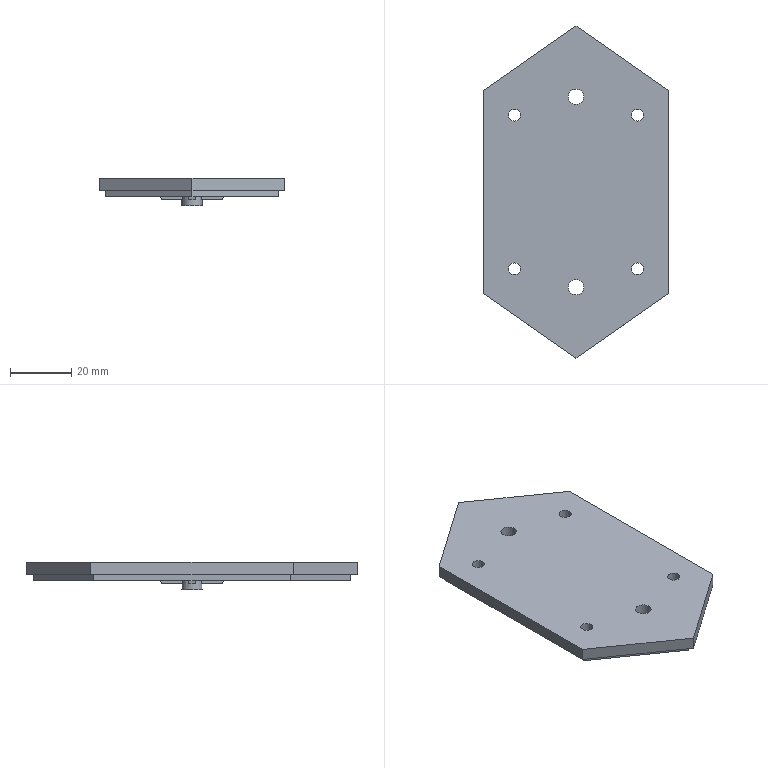Component | NX | BASE_PLATE | 1 solid | 48 faces | volume 21864 mm3 | plane 40 | cylinder 8 | commonest cylinder face diameters 3.903 x4 5 x2 6.6 x1 3 x1